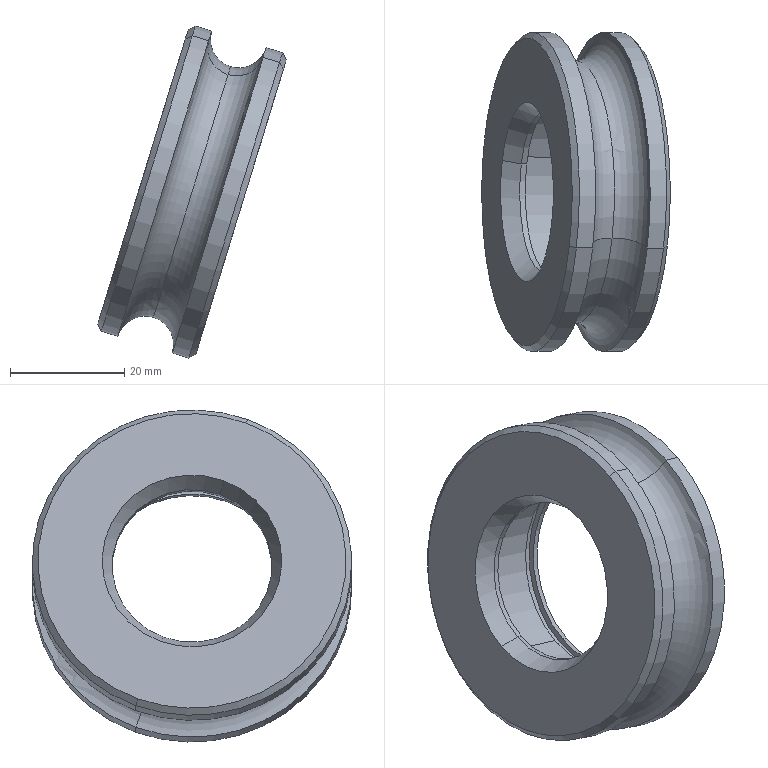Component | SolidWorks | DriveDevice-1_GuideWheelHub-1 | 1 solid | 27 faces | box 33.05 x 56 x 58.23 mm | volume 21349 mm3 | cylinder 12 | cone 6 | plane 5 | torus 4 | commonest cylinder face diameters 56 x4 35 x4 37 x2 28 x2
build123d program:
from build123d import *


with BuildPart() as part:
    # Sketch1 → Revolve1 (revolve)
    with BuildSketch(Plane(origin=(0, 0, 0), x_dir=(0, 0, -1), z_dir=(1, 0, 0)), mode=Mode.PRIVATE) as revolve1_sk:
        with BuildLine():
            Line((2.985, 14), (3.985, 14))
            Line((3.985, 14), (3.985, 17.5))
            Line((3.985, 17.5), (14.985, 17.5))
            Line((14.985, 17.5), (14.985, 18.5))
            Line((14.985, 18.5), (16.985, 18.5))
            Line((16.985, 18.5), (16.985, 17.5))
            Line((16.985, 17.5), (17.985, 17.5))
            Line((17.985, 17.5), (17.985, 27))
            Line((17.985, 27), (16.985, 28))
            Line((16.985, 28), (13.992, 28))
            ThreePointArc((13.992, 28), (8.992, 23), (3.992, 28))
            Line((3.992, 28), (1, 28))
            Line((1, 28), (0, 27))
            Line((0, 27), (0, 15.75))
            Line((0, 15.75), (2.985, 14))
        make_face()
    revolve(revolve1_sk.sketch.rotate(Axis((0, 0, 0), (0, 0, -1)), 90), axis=Axis((0, 0, 0), (0, 0, -1)))


solid = part.part

# Placed as in the assembly
solid = solid.moved(Location((-214.709, 15, 17.054), (0, -72.922, 83.044)))
STEP:
#1=COLOUR_RGB('',0.7922,0.8196,0.9333);
#2=FILL_AREA_STYLE_COLOUR('',#1);
#3=FILL_AREA_STYLE('',(#2));
#4=SURFACE_STYLE_FILL_AREA(#3);
#5=SURFACE_SIDE_STYLE('',(#4));
#6=SURFACE_STYLE_USAGE(.BOTH.,#5);
#7=PRESENTATION_STYLE_ASSIGNMENT((#6));
#8=CARTESIAN_POINT('',(-8.606,0.9787,-0.361));
#9=VERTEX_POINT('',#8);
#10=CARTESIAN_POINT('',(-8.364,0.9094,-0.2427));
#11=VERTEX_POINT('',#10);
#12=CARTESIAN_POINT('',(-8.418,0.9787,-0.4188));
#13=DIRECTION('',(0.1034,0.936,0.3366));
#14=DIRECTION('',(0.,-0.3384,0.941));
#15=AXIS2_PLACEMENT_3D('',#12,#13,#14);
#16=CIRCLE('',#15,0.1969);
#17=EDGE_CURVE('',#9,#11,#16,.T.);
#18=ORIENTED_EDGE('',*,*,#17,.T.);
#19=CARTESIAN_POINT('',(-7.866,0.2717,1.378));
#20=VERTEX_POINT('',#19);
#21=CARTESIAN_POINT('',(-8.115,0.5906,0.5675));
#22=DIRECTION('',(-0.9559,-0.,0.2937));
#23=DIRECTION('',(0.2937,0.,0.9559));
#24=AXIS2_PLACEMENT_3D('',#21,#22,#23);
#25=CIRCLE('',#24,0.9055);
#26=EDGE_CURVE('',#11,#20,#25,.T.);
#27=ORIENTED_EDGE('',*,*,#26,.T.);
#28=CARTESIAN_POINT('',(-8.,0.2024,1.612));
#29=VERTEX_POINT('',#28);
#30=CARTESIAN_POINT('',(-7.812,0.2024,1.554));
#31=DIRECTION('',(-0.1034,-0.936,-0.3366));
#32=DIRECTION('',(0.,0.3384,-0.941));
#33=AXIS2_PLACEMENT_3D('',#30,#31,#32);
#34=CIRCLE('',#33,0.1969);
#35=EDGE_CURVE('',#29,#20,#34,.T.);
#36=ORIENTED_EDGE('',*,*,#35,.F.);
#37=CARTESIAN_POINT('',(-8.303,0.5906,0.6253));
#38=DIRECTION('',(-0.9559,-0.,0.2937));
#39=DIRECTION('',(-0.2749,0.3521,-0.8947));
#40=AXIS2_PLACEMENT_3D('',#37,#38,#39);
#41=CIRCLE('',#40,1.102);
#42=EDGE_CURVE('',#9,#29,#41,.T.);
#43=ORIENTED_EDGE('',*,*,#42,.F.);
#44=EDGE_LOOP('',(#18,#27,#36,#43));
#45=FACE_OUTER_BOUND('',#44,.T.);
#46=CARTESIAN_POINT('',(-8.115,0.5906,0.5675));
#47=DIRECTION('',(-0.9559,-0.,0.2937));
#48=DIRECTION('',(-0.2749,0.3521,-0.8947));
#49=AXIS2_PLACEMENT_3D('',#46,#47,#48);
#50=TOROIDAL_SURFACE('',#49,1.102,0.1969);
#51=ADVANCED_FACE('',(#45),#50,.F.);
#52=ORIENTED_EDGE('',*,*,#35,.T.);
#53=CARTESIAN_POINT('',(-8.115,0.5906,0.5675));
#54=DIRECTION('',(-0.9559,-0.,0.2937));
#55=DIRECTION('',(0.2937,0.,0.9559));
#56=AXIS2_PLACEMENT_3D('',#53,#54,#55);
#57=CIRCLE('',#56,0.9055);
#58=EDGE_CURVE('',#20,#11,#57,.T.);
#59=ORIENTED_EDGE('',*,*,#58,.T.);
#60=ORIENTED_EDGE('',*,*,#17,.F.);
#61=CARTESIAN_POINT('',(-8.303,0.5906,0.6253));
#62=DIRECTION('',(-0.9559,-0.,0.2937));
#63=DIRECTION('',(-0.2749,0.3521,-0.8947));
#64=AXIS2_PLACEMENT_3D('',#61,#62,#63);
#65=CIRCLE('',#64,1.102);
#66=EDGE_CURVE('',#29,#9,#65,.T.);
#67=ORIENTED_EDGE('',*,*,#66,.F.);
#68=EDGE_LOOP('',(#52,#59,#60,#67));
#69=FACE_OUTER_BOUND('',#68,.T.);
#70=CARTESIAN_POINT('',(-8.115,0.5906,0.5675));
#71=DIRECTION('',(-0.9559,-0.,0.2937));
#72=DIRECTION('',(-0.2749,0.3521,-0.8947));
#73=AXIS2_PLACEMENT_3D('',#70,#71,#72);
#74=TOROIDAL_SURFACE('',#73,1.102,0.1969);
#75=ADVANCED_FACE('',(#69),#74,.F.);
#76=CARTESIAN_POINT('',(-8.745,0.9648,-0.2796));
#77=VERTEX_POINT('',#76);
#78=CARTESIAN_POINT('',(-8.161,0.2163,1.622));
#79=VERTEX_POINT('',#78);
#80=CARTESIAN_POINT('',(-8.453,0.5906,0.6714));
#81=DIRECTION('',(-0.9559,-0.,0.2937));
#82=DIRECTION('',(-0.2749,0.3521,-0.8947));
#83=AXIS2_PLACEMENT_3D('',#80,#81,#82);
#84=CIRCLE('',#83,1.063);
#85=EDGE_CURVE('',#77,#79,#84,.T.);
#86=ORIENTED_EDGE('',*,*,#85,.F.);
#87=CARTESIAN_POINT('',(-8.718,0.9787,-0.3264));
#88=VERTEX_POINT('',#87);
#89=CARTESIAN_POINT('',(-8.718,0.9787,-0.3264));
#90=DIRECTION('',(0.4816,0.249,-0.8403));
#91=VECTOR('',#90,39.37);
#92=LINE('',#89,#91);
#93=EDGE_CURVE('',#77,#88,#92,.T.);
#94=ORIENTED_EDGE('',*,*,#93,.T.);
#95=CARTESIAN_POINT('',(-8.112,0.2024,1.646));
#96=VERTEX_POINT('',#95);
#97=CARTESIAN_POINT('',(-8.415,0.5906,0.6599));
#98=DIRECTION('',(-0.9559,-0.,0.2937));
#99=DIRECTION('',(-0.2749,0.3521,-0.8947));
#100=AXIS2_PLACEMENT_3D('',#97,#98,#99);
#101=CIRCLE('',#100,1.102);
#102=EDGE_CURVE('',#88,#96,#101,.T.);
#103=ORIENTED_EDGE('',*,*,#102,.T.);
#104=CARTESIAN_POINT('',(-8.112,0.2024,1.646));
#105=DIRECTION('',(0.8703,-0.249,0.425));
#106=VECTOR('',#105,39.37);
#107=LINE('',#104,#106);
#108=EDGE_CURVE('',#79,#96,#107,.T.);
#109=ORIENTED_EDGE('',*,*,#108,.F.);
#110=EDGE_LOOP('',(#86,#94,#103,#109));
#111=FACE_OUTER_BOUND('',#110,.T.);
#112=CARTESIAN_POINT('',(-8.415,0.5906,0.6599));
#113=DIRECTION('',(0.9559,0.,-0.2937));
#114=DIRECTION('',(0.2749,-0.3521,0.8947));
#115=AXIS2_PLACEMENT_3D('',#112,#113,#114);
#116=CONICAL_SURFACE('',#115,1.102,0.7854);
#117=ADVANCED_FACE('',(#111),#116,.T.);
#118=ORIENTED_EDGE('',*,*,#42,.T.);
#119=CARTESIAN_POINT('',(-8.15,0.2024,1.658));
#120=DIRECTION('',(-0.9559,-0.,0.2937));
#121=VECTOR('',#120,39.37);
#122=LINE('',#119,#121);
#123=EDGE_CURVE('',#29,#96,#122,.T.);
#124=ORIENTED_EDGE('',*,*,#123,.T.);
#125=ORIENTED_EDGE('',*,*,#102,.F.);
#126=CARTESIAN_POINT('',(-8.756,0.9787,-0.3148));
#127=DIRECTION('',(-0.9559,-0.,0.2937));
#128=VECTOR('',#127,39.37);
#129=LINE('',#126,#128);
#130=EDGE_CURVE('',#9,#88,#129,.T.);
#131=ORIENTED_EDGE('',*,*,#130,.F.);
#132=EDGE_LOOP('',(#118,#124,#125,#131));
#133=FACE_OUTER_BOUND('',#132,.T.);
#134=CARTESIAN_POINT('',(-8.453,0.5906,0.6714));
#135=DIRECTION('',(-0.9559,-0.,0.2937));
#136=DIRECTION('',(-0.2749,0.3521,-0.8947));
#137=AXIS2_PLACEMENT_3D('',#134,#135,#136);
#138=CYLINDRICAL_SURFACE('',#137,1.102);
#139=ADVANCED_FACE('',(#133),#138,.T.);
#140=ORIENTED_EDGE('',*,*,#58,.F.);
#141=CARTESIAN_POINT('',(-7.624,0.2024,1.496));
#142=VERTEX_POINT('',#141);
#143=CARTESIAN_POINT('',(-7.812,0.2024,1.554));
#144=DIRECTION('',(-0.1034,-0.936,-0.3366));
#145=DIRECTION('',(0.,0.3384,-0.941));
#146=AXIS2_PLACEMENT_3D('',#143,#144,#145);
#147=CIRCLE('',#146,0.1969);
#148=EDGE_CURVE('',#20,#142,#147,.T.);
#149=ORIENTED_EDGE('',*,*,#148,.T.);
#150=CARTESIAN_POINT('',(-8.23,0.9787,-0.4766));
#151=VERTEX_POINT('',#150);
#152=CARTESIAN_POINT('',(-7.927,0.5906,0.5097));
#153=DIRECTION('',(-0.9559,-0.,0.2937));
#154=DIRECTION('',(-0.2749,0.3521,-0.8947));
#155=AXIS2_PLACEMENT_3D('',#152,#153,#154);
#156=CIRCLE('',#155,1.102);
#157=EDGE_CURVE('',#142,#151,#156,.T.);
#158=ORIENTED_EDGE('',*,*,#157,.T.);
#159=CARTESIAN_POINT('',(-8.418,0.9787,-0.4188));
#160=DIRECTION('',(0.1034,0.936,0.3366));
#161=DIRECTION('',(0.,-0.3384,0.941));
#162=AXIS2_PLACEMENT_3D('',#159,#160,#161);
#163=CIRCLE('',#162,0.1969);
#164=EDGE_CURVE('',#11,#151,#163,.T.);
#165=ORIENTED_EDGE('',*,*,#164,.F.);
#166=EDGE_LOOP('',(#140,#149,#158,#165));
#167=FACE_OUTER_BOUND('',#166,.T.);
#168=CARTESIAN_POINT('',(-8.115,0.5906,0.5675));
#169=DIRECTION('',(-0.9559,-0.,0.2937));
#170=DIRECTION('',(-0.2749,0.3521,-0.8947));
#171=AXIS2_PLACEMENT_3D('',#168,#169,#170);
#172=TOROIDAL_SURFACE('',#171,1.102,0.1969);
#173=ADVANCED_FACE('',(#167),#172,.F.);
#174=CARTESIAN_POINT('',(-8.117,0.9787,-0.5112));
#175=VERTEX_POINT('',#174);
#176=CARTESIAN_POINT('',(-7.511,0.2024,1.461));
#177=VERTEX_POINT('',#176);
#178=CARTESIAN_POINT('',(-7.814,0.5906,0.4751));
#179=DIRECTION('',(-0.9559,-0.,0.2937));
#180=DIRECTION('',(-0.2749,0.3521,-0.8947));
#181=AXIS2_PLACEMENT_3D('',#178,#179,#180);
#182=CIRCLE('',#181,1.102);
#183=EDGE_CURVE('',#175,#177,#182,.T.);
#184=ORIENTED_EDGE('',*,*,#183,.T.);
#185=CARTESIAN_POINT('',(-8.15,0.2024,1.658));
#186=DIRECTION('',(-0.9559,-0.,0.2937));
#187=VECTOR('',#186,39.37);
#188=LINE('',#185,#187);
#189=EDGE_CURVE('',#177,#142,#188,.T.);
#190=ORIENTED_EDGE('',*,*,#189,.T.);
#191=CARTESIAN_POINT('',(-7.927,0.5906,0.5097));
#192=DIRECTION('',(-0.9559,-0.,0.2937));
#193=DIRECTION('',(-0.2749,0.3521,-0.8947));
#194=AXIS2_PLACEMENT_3D('',#191,#192,#193);
#195=CIRCLE('',#194,1.102);
#196=EDGE_CURVE('',#151,#142,#195,.T.);
#197=ORIENTED_EDGE('',*,*,#196,.F.);
#198=CARTESIAN_POINT('',(-8.756,0.9787,-0.3148));
#199=DIRECTION('',(-0.9559,-0.,0.2937));
#200=VECTOR('',#199,39.37);
#201=LINE('',#198,#200);
#202=EDGE_CURVE('',#175,#151,#201,.T.);
#203=ORIENTED_EDGE('',*,*,#202,.F.);
#204=EDGE_LOOP('',(#184,#190,#197,#203));
#205=FACE_OUTER_BOUND('',#204,.T.);
#206=CARTESIAN_POINT('',(-8.453,0.5906,0.6714));
#207=DIRECTION('',(-0.9559,-0.,0.2937));
#208=DIRECTION('',(-0.2749,0.3521,-0.8947));
#209=AXIS2_PLACEMENT_3D('',#206,#207,#208);
#210=CYLINDRICAL_SURFACE('',#209,1.102);
#211=ADVANCED_FACE('',(#205),#210,.T.);
#212=CARTESIAN_POINT('',(-8.068,0.9648,-0.4876));
#213=VERTEX_POINT('',#212);
#214=CARTESIAN_POINT('',(-7.484,0.2163,1.415));
#215=VERTEX_POINT('',#214);
#216=CARTESIAN_POINT('',(-7.776,0.5906,0.4635));
#217=DIRECTION('',(-0.9559,-0.,0.2937));
#218=DIRECTION('',(-0.2749,0.3521,-0.8947));
#219=AXIS2_PLACEMENT_3D('',#216,#217,#218);
#220=CIRCLE('',#219,1.063);
#221=EDGE_CURVE('',#213,#215,#220,.T.);
#222=ORIENTED_EDGE('',*,*,#221,.T.);
#223=CARTESIAN_POINT('',(-7.484,0.2163,1.415));
#224=DIRECTION('',(-0.4816,-0.249,0.8403));
#225=VECTOR('',#224,39.37);
#226=LINE('',#223,#225);
#227=EDGE_CURVE('',#215,#177,#226,.T.);
#228=ORIENTED_EDGE('',*,*,#227,.T.);
#229=ORIENTED_EDGE('',*,*,#183,.F.);
#230=CARTESIAN_POINT('',(-8.068,0.9648,-0.4876));
#231=DIRECTION('',(-0.8703,0.249,-0.425));
#232=VECTOR('',#231,39.37);
#233=LINE('',#230,#232);
#234=EDGE_CURVE('',#213,#175,#233,.T.);
#235=ORIENTED_EDGE('',*,*,#234,.F.);
#236=EDGE_LOOP('',(#222,#228,#229,#235));
#237=FACE_OUTER_BOUND('',#236,.T.);
#238=CARTESIAN_POINT('',(-7.776,0.5906,0.4635));
#239=DIRECTION('',(-0.9559,-0.,0.2937));
#240=DIRECTION('',(-0.2749,0.3521,-0.8947));
#241=AXIS2_PLACEMENT_3D('',#238,#239,#240);
#242=CONICAL_SURFACE('',#241,1.063,0.7854);
#243=ADVANCED_FACE('',(#237),#242,.T.);
#244=CARTESIAN_POINT('',(-7.587,0.348,1.08));
#245=VERTEX_POINT('',#244);
#246=CARTESIAN_POINT('',(-7.966,0.8331,-0.1529));
#247=VERTEX_POINT('',#246);
#248=CARTESIAN_POINT('',(-7.776,0.5906,0.4635));
#249=DIRECTION('',(-0.9559,-0.,0.2937));
#250=DIRECTION('',(-0.2749,0.3521,-0.8947));
#251=AXIS2_PLACEMENT_3D('',#248,#249,#250);
#252=CIRCLE('',#251,0.689);
#253=EDGE_CURVE('',#245,#247,#252,.T.);
#254=ORIENTED_EDGE('',*,*,#253,.F.);
#255=CARTESIAN_POINT('',(-7.625,0.348,1.091));
#256=VERTEX_POINT('',#255);
#257=CARTESIAN_POINT('',(-8.264,0.348,1.288));
#258=DIRECTION('',(-0.9559,-0.,0.2937));
#259=VECTOR('',#258,39.37);
#260=LINE('',#257,#259);
#261=EDGE_CURVE('',#245,#256,#260,.T.);
#262=ORIENTED_EDGE('',*,*,#261,.T.);
#263=CARTESIAN_POINT('',(-8.003,0.8331,-0.1414));
#264=VERTEX_POINT('',#263);
#265=CARTESIAN_POINT('',(-7.814,0.5906,0.4751));
#266=DIRECTION('',(-0.9559,-0.,0.2937));
#267=DIRECTION('',(-0.2749,0.3521,-0.8947));
#268=AXIS2_PLACEMENT_3D('',#265,#266,#267);
#269=CIRCLE('',#268,0.689);
#270=EDGE_CURVE('',#256,#264,#269,.T.);
#271=ORIENTED_EDGE('',*,*,#270,.T.);
#272=CARTESIAN_POINT('',(-8.642,0.8331,0.05501));
#273=DIRECTION('',(-0.9559,-0.,0.2937));
#274=VECTOR('',#273,39.37);
#275=LINE('',#272,#274);
#276=EDGE_CURVE('',#247,#264,#275,.T.);
#277=ORIENTED_EDGE('',*,*,#276,.F.);
#278=EDGE_LOOP('',(#254,#262,#271,#277));
#279=FACE_OUTER_BOUND('',#278,.T.);
#280=CARTESIAN_POINT('',(-8.453,0.5906,0.6714));
#281=DIRECTION('',(-0.9559,-0.,0.2937));
#282=DIRECTION('',(-0.2749,0.3521,-0.8947));
#283=AXIS2_PLACEMENT_3D('',#280,#281,#282);
#284=CYLINDRICAL_SURFACE('',#283,0.689);
#285=ADVANCED_FACE('',(#279),#284,.F.);
#286=CARTESIAN_POINT('',(-7.614,0.3341,1.127));
#287=VERTEX_POINT('',#286);
#288=CARTESIAN_POINT('',(-8.014,0.847,-0.1766));
#289=VERTEX_POINT('',#288);
#290=CARTESIAN_POINT('',(-7.814,0.5906,0.4751));
#291=DIRECTION('',(-0.9559,-0.,0.2937));
#292=DIRECTION('',(-0.2749,0.3521,-0.8947));
#293=AXIS2_PLACEMENT_3D('',#290,#291,#292);
#294=CIRCLE('',#293,0.7283);
#295=EDGE_CURVE('',#287,#289,#294,.T.);
#296=ORIENTED_EDGE('',*,*,#295,.F.);
#297=CARTESIAN_POINT('',(-7.689,0.3341,1.15));
#298=VERTEX_POINT('',#297);
#299=CARTESIAN_POINT('',(-8.253,0.3341,1.323));
#300=DIRECTION('',(-0.9559,-0.,0.2937));
#301=VECTOR('',#300,39.37);
#302=LINE('',#299,#301);
#303=EDGE_CURVE('',#287,#298,#302,.T.);
#304=ORIENTED_EDGE('',*,*,#303,.T.);
#305=CARTESIAN_POINT('',(-8.089,0.847,-0.1535));
#306=VERTEX_POINT('',#305);
#307=CARTESIAN_POINT('',(-7.889,0.5906,0.4982));
#308=DIRECTION('',(-0.9559,-0.,0.2937));
#309=DIRECTION('',(-0.2749,0.3521,-0.8947));
#310=AXIS2_PLACEMENT_3D('',#307,#308,#309);
#311=CIRCLE('',#310,0.7283);
#312=EDGE_CURVE('',#298,#306,#311,.T.);
#313=ORIENTED_EDGE('',*,*,#312,.T.);
#314=CARTESIAN_POINT('',(-8.653,0.847,0.01979));
#315=DIRECTION('',(-0.9559,-0.,0.2937));
#316=VECTOR('',#315,39.37);
#317=LINE('',#314,#316);
#318=EDGE_CURVE('',#289,#306,#317,.T.);
#319=ORIENTED_EDGE('',*,*,#318,.F.);
#320=EDGE_LOOP('',(#296,#304,#313,#319));
#321=FACE_OUTER_BOUND('',#320,.T.);
#322=CARTESIAN_POINT('',(-8.453,0.5906,0.6714));
#323=DIRECTION('',(-0.9559,-0.,0.2937));
#324=DIRECTION('',(-0.2749,0.3521,-0.8947));
#325=AXIS2_PLACEMENT_3D('',#322,#323,#324);
#326=CYLINDRICAL_SURFACE('',#325,0.7283);
#327=ADVANCED_FACE('',(#321),#326,.F.);
#328=CARTESIAN_POINT('',(-7.7,0.348,1.115));
#329=VERTEX_POINT('',#328);
#330=CARTESIAN_POINT('',(-8.079,0.8331,-0.1182));
#331=VERTEX_POINT('',#330);
#332=CARTESIAN_POINT('',(-7.889,0.5906,0.4982));
#333=DIRECTION('',(-0.9559,-0.,0.2937));
#334=DIRECTION('',(-0.2749,0.3521,-0.8947));
#335=AXIS2_PLACEMENT_3D('',#332,#333,#334);
#336=CIRCLE('',#335,0.689);
#337=EDGE_CURVE('',#329,#331,#336,.T.);
#338=ORIENTED_EDGE('',*,*,#337,.F.);
#339=CARTESIAN_POINT('',(-8.114,0.348,1.242));
#340=VERTEX_POINT('',#339);
#341=CARTESIAN_POINT('',(-8.264,0.348,1.288));
#342=DIRECTION('',(-0.9559,-0.,0.2937));
#343=VECTOR('',#342,39.37);
#344=LINE('',#341,#343);
#345=EDGE_CURVE('',#329,#340,#344,.T.);
#346=ORIENTED_EDGE('',*,*,#345,.T.);
#347=CARTESIAN_POINT('',(-8.493,0.8331,0.008942));
#348=VERTEX_POINT('',#347);
#349=CARTESIAN_POINT('',(-8.303,0.5906,0.6254));
#350=DIRECTION('',(-0.9559,-0.,0.2937));
#351=DIRECTION('',(-0.2749,0.3521,-0.8947));
#352=AXIS2_PLACEMENT_3D('',#349,#350,#351);
#353=CIRCLE('',#352,0.689);
#354=EDGE_CURVE('',#340,#348,#353,.T.);
#355=ORIENTED_EDGE('',*,*,#354,.T.);
#356=CARTESIAN_POINT('',(-8.642,0.8331,0.05501));
#357=DIRECTION('',(-0.9559,-0.,0.2937));
#358=VECTOR('',#357,39.37);
#359=LINE('',#356,#358);
#360=EDGE_CURVE('',#331,#348,#359,.T.);
#361=ORIENTED_EDGE('',*,*,#360,.F.);
#362=EDGE_LOOP('',(#338,#346,#355,#361));
#363=FACE_OUTER_BOUND('',#362,.T.);
#364=CARTESIAN_POINT('',(-8.453,0.5906,0.6714));
#365=DIRECTION('',(-0.9559,-0.,0.2937));
#366=DIRECTION('',(-0.2749,0.3521,-0.8947));
#367=AXIS2_PLACEMENT_3D('',#364,#365,#366);
#368=CYLINDRICAL_SURFACE('',#367,0.689);
#369=ADVANCED_FACE('',(#363),#368,.F.);
#370=CARTESIAN_POINT('',(-8.152,0.3965,1.119));
#371=VERTEX_POINT('',#370);
#372=CARTESIAN_POINT('',(-8.455,0.7846,0.1322));
#373=VERTEX_POINT('',#372);
#374=CARTESIAN_POINT('',(-8.303,0.5906,0.6254));
#375=DIRECTION('',(-0.9559,-0.,0.2937));
#376=DIRECTION('',(-0.2749,0.3521,-0.8947));
#377=AXIS2_PLACEMENT_3D('',#374,#375,#376);
#378=CIRCLE('',#377,0.5512);
#379=EDGE_CURVE('',#371,#373,#378,.T.);
#380=ORIENTED_EDGE('',*,*,#379,.F.);
#381=CARTESIAN_POINT('',(-8.189,0.3965,1.13));
#382=VERTEX_POINT('',#381);
#383=CARTESIAN_POINT('',(-8.302,0.3965,1.165));
#384=DIRECTION('',(-0.9559,-0.,0.2937));
#385=VECTOR('',#384,39.37);
#386=LINE('',#383,#385);
#387=EDGE_CURVE('',#371,#382,#386,.T.);
#388=ORIENTED_EDGE('',*,*,#387,.T.);
#389=CARTESIAN_POINT('',(-8.492,0.7846,0.1438));
#390=VERTEX_POINT('',#389);
#391=CARTESIAN_POINT('',(-8.341,0.5906,0.6369));
#392=DIRECTION('',(-0.9559,-0.,0.2937));
#393=DIRECTION('',(-0.2749,0.3521,-0.8947));
#394=AXIS2_PLACEMENT_3D('',#391,#392,#393);
#395=CIRCLE('',#394,0.5512);
#396=EDGE_CURVE('',#382,#390,#395,.T.);
#397=ORIENTED_EDGE('',*,*,#396,.T.);
#398=CARTESIAN_POINT('',(-8.605,0.7846,0.1783));
#399=DIRECTION('',(-0.9559,-0.,0.2937));
#400=VECTOR('',#399,39.37);
#401=LINE('',#398,#400);
#402=EDGE_CURVE('',#373,#390,#401,.T.);
#403=ORIENTED_EDGE('',*,*,#402,.F.);
#404=EDGE_LOOP('',(#380,#388,#397,#403));
#405=FACE_OUTER_BOUND('',#404,.T.);
#406=CARTESIAN_POINT('',(-8.453,0.5906,0.6714));
#407=DIRECTION('',(-0.9559,-0.,0.2937));
#408=DIRECTION('',(-0.2749,0.3521,-0.8947));
#409=AXIS2_PLACEMENT_3D('',#406,#407,#408);
#410=CYLINDRICAL_SURFACE('',#409,0.5512);
#411=ADVANCED_FACE('',(#405),#410,.F.);
#412=ORIENTED_EDGE('',*,*,#396,.F.);
#413=CARTESIAN_POINT('',(-8.283,0.3722,1.226));
#414=VERTEX_POINT('',#413);
#415=CARTESIAN_POINT('',(-8.283,0.3722,1.226));
#416=DIRECTION('',(-0.6856,-0.1781,0.7059));
#417=VECTOR('',#416,39.37);
#418=LINE('',#415,#417);
#419=EDGE_CURVE('',#382,#414,#418,.T.);
#420=ORIENTED_EDGE('',*,*,#419,.T.);
#421=CARTESIAN_POINT('',(-8.624,0.8089,0.1167));
#422=VERTEX_POINT('',#421);
#423=CARTESIAN_POINT('',(-8.453,0.5906,0.6714));
#424=DIRECTION('',(-0.9559,-0.,0.2937));
#425=DIRECTION('',(-0.2749,0.3521,-0.8947));
#426=AXIS2_PLACEMENT_3D('',#423,#424,#425);
#427=CIRCLE('',#426,0.6201);
#428=EDGE_CURVE('',#414,#422,#427,.T.);
#429=ORIENTED_EDGE('',*,*,#428,.T.);
#430=CARTESIAN_POINT('',(-8.624,0.8089,0.1167));
#431=DIRECTION('',(-0.9636,0.1781,-0.1992));
#432=VECTOR('',#431,39.37);
#433=LINE('',#430,#432);
#434=EDGE_CURVE('',#390,#422,#433,.T.);
#435=ORIENTED_EDGE('',*,*,#434,.F.);
#436=EDGE_LOOP('',(#412,#420,#429,#435));
#437=FACE_OUTER_BOUND('',#436,.T.);
#438=CARTESIAN_POINT('',(-8.453,0.5906,0.6714));
#439=DIRECTION('',(-0.9559,-0.,0.2937));
#440=DIRECTION('',(-0.2749,0.3521,-0.8947));
#441=AXIS2_PLACEMENT_3D('',#438,#439,#440);
#442=CONICAL_SURFACE('',#441,0.6201,0.5303);
#443=ADVANCED_FACE('',(#437),#442,.F.);
#444=ORIENTED_EDGE('',*,*,#419,.F.);
#445=CARTESIAN_POINT('',(-8.341,0.5906,0.6369));
#446=DIRECTION('',(-0.9559,-0.,0.2937));
#447=DIRECTION('',(-0.2749,0.3521,-0.8947));
#448=AXIS2_PLACEMENT_3D('',#445,#446,#447);
#449=CIRCLE('',#448,0.5512);
#450=EDGE_CURVE('',#390,#382,#449,.T.);
#451=ORIENTED_EDGE('',*,*,#450,.F.);
#452=ORIENTED_EDGE('',*,*,#434,.T.);
#453=CARTESIAN_POINT('',(-8.453,0.5906,0.6714));
#454=DIRECTION('',(-0.9559,-0.,0.2937));
#455=DIRECTION('',(-0.2749,0.3521,-0.8947));
#456=AXIS2_PLACEMENT_3D('',#453,#454,#455);
#457=CIRCLE('',#456,0.6201);
#458=EDGE_CURVE('',#422,#414,#457,.T.);
#459=ORIENTED_EDGE('',*,*,#458,.T.);
#460=EDGE_LOOP('',(#444,#451,#452,#459));
#461=FACE_OUTER_BOUND('',#460,.T.);
#462=CARTESIAN_POINT('',(-8.453,0.5906,0.6714));
#463=DIRECTION('',(-0.9559,-0.,0.2937));
#464=DIRECTION('',(-0.2749,0.3521,-0.8947));
#465=AXIS2_PLACEMENT_3D('',#462,#463,#464);
#466=CONICAL_SURFACE('',#465,0.6201,0.5303);
#467=ADVANCED_FACE('',(#461),#466,.F.);
#468=ORIENTED_EDGE('',*,*,#387,.F.);
#469=CARTESIAN_POINT('',(-8.303,0.5906,0.6254));
#470=DIRECTION('',(-0.9559,-0.,0.2937));
#471=DIRECTION('',(-0.2749,0.3521,-0.8947));
#472=AXIS2_PLACEMENT_3D('',#469,#470,#471);
#473=CIRCLE('',#472,0.5512);
#474=EDGE_CURVE('',#373,#371,#473,.T.);
#475=ORIENTED_EDGE('',*,*,#474,.F.);
#476=ORIENTED_EDGE('',*,*,#402,.T.);
#477=ORIENTED_EDGE('',*,*,#450,.T.);
#478=EDGE_LOOP('',(#468,#475,#476,#477));
#479=FACE_OUTER_BOUND('',#478,.T.);
#480=CARTESIAN_POINT('',(-8.453,0.5906,0.6714));
#481=DIRECTION('',(-0.9559,-0.,0.2937));
#482=DIRECTION('',(-0.2749,0.3521,-0.8947));
#483=AXIS2_PLACEMENT_3D('',#480,#481,#482);
#484=CYLINDRICAL_SURFACE('',#483,0.5512);
#485=ADVANCED_FACE('',(#479),#484,.F.);
#486=CARTESIAN_POINT('',(-8.303,0.5906,0.6254));
#487=DIRECTION('',(-0.9559,-0.,0.2937));
#488=DIRECTION('',(-0.2749,0.3521,-0.8947));
#489=AXIS2_PLACEMENT_3D('',#486,#487,#488);
#490=CIRCLE('',#489,0.689);
#491=EDGE_CURVE('',#348,#340,#490,.T.);
#492=ORIENTED_EDGE('',*,*,#491,.F.);
#493=ORIENTED_EDGE('',*,*,#354,.F.);
#494=EDGE_LOOP('',(#492,#493));
#495=FACE_OUTER_BOUND('',#494,.T.);
#496=ORIENTED_EDGE('',*,*,#474,.T.);
#497=ORIENTED_EDGE('',*,*,#379,.T.);
#498=EDGE_LOOP('',(#496,#497));
#499=FACE_BOUND('',#498,.T.);
#500=CARTESIAN_POINT('',(-8.36,0.07467,0.4399));
#501=DIRECTION('',(-0.9559,-0.,0.2937));
#502=DIRECTION('',(-0.2749,0.3521,-0.8947));
#503=AXIS2_PLACEMENT_3D('',#500,#501,#502);
#504=PLANE('',#503);
#505=ADVANCED_FACE('',(#495,#499),#504,.F.);
#506=ORIENTED_EDGE('',*,*,#345,.F.);
#507=CARTESIAN_POINT('',(-7.889,0.5906,0.4982));
#508=DIRECTION('',(-0.9559,-0.,0.2937));
#509=DIRECTION('',(-0.2749,0.3521,-0.8947));
#510=AXIS2_PLACEMENT_3D('',#507,#508,#509);
#511=CIRCLE('',#510,0.689);
#512=EDGE_CURVE('',#331,#329,#511,.T.);
#513=ORIENTED_EDGE('',*,*,#512,.F.);
#514=ORIENTED_EDGE('',*,*,#360,.T.);
#515=ORIENTED_EDGE('',*,*,#491,.T.);
#516=EDGE_LOOP('',(#506,#513,#514,#515));
#517=FACE_OUTER_BOUND('',#516,.T.);
#518=CARTESIAN_POINT('',(-8.453,0.5906,0.6714));
#519=DIRECTION('',(-0.9559,-0.,0.2937));
#520=DIRECTION('',(-0.2749,0.3521,-0.8947));
#521=AXIS2_PLACEMENT_3D('',#518,#519,#520);
#522=CYLINDRICAL_SURFACE('',#521,0.689);
#523=ADVANCED_FACE('',(#517),#522,.F.);
#524=CARTESIAN_POINT('',(-7.889,0.5906,0.4982));
#525=DIRECTION('',(-0.9559,-0.,0.2937));
#526=DIRECTION('',(-0.2749,0.3521,-0.8947));
#527=AXIS2_PLACEMENT_3D('',#524,#525,#526);
#528=CIRCLE('',#527,0.7283);
#529=EDGE_CURVE('',#306,#298,#528,.T.);
#530=ORIENTED_EDGE('',*,*,#529,.F.);
#531=ORIENTED_EDGE('',*,*,#312,.F.);
#532=EDGE_LOOP('',(#530,#531));
#533=FACE_OUTER_BOUND('',#532,.T.);
#534=ORIENTED_EDGE('',*,*,#512,.T.);
#535=ORIENTED_EDGE('',*,*,#337,.T.);
#536=EDGE_LOOP('',(#534,#535));
#537=FACE_BOUND('',#536,.T.);
#538=CARTESIAN_POINT('',(-7.96,-0.05431,0.2663));
#539=DIRECTION('',(-0.9559,-0.,0.2937));
#540=DIRECTION('',(-0.2749,0.3521,-0.8947));
#541=AXIS2_PLACEMENT_3D('',#538,#539,#540);
#542=PLANE('',#541);
#543=ADVANCED_FACE('',(#533,#537),#542,.F.);
#544=ORIENTED_EDGE('',*,*,#303,.F.);
#545=CARTESIAN_POINT('',(-7.814,0.5906,0.4751));
#546=DIRECTION('',(-0.9559,-0.,0.2937));
#547=DIRECTION('',(-0.2749,0.3521,-0.8947));
#548=AXIS2_PLACEMENT_3D('',#545,#546,#547);
#549=CIRCLE('',#548,0.7283);
#550=EDGE_CURVE('',#289,#287,#549,.T.);
#551=ORIENTED_EDGE('',*,*,#550,.F.);
#552=ORIENTED_EDGE('',*,*,#318,.T.);
#553=ORIENTED_EDGE('',*,*,#529,.T.);
#554=EDGE_LOOP('',(#544,#551,#552,#553));
#555=FACE_OUTER_BOUND('',#554,.T.);
#556=CARTESIAN_POINT('',(-8.453,0.5906,0.6714));
#557=DIRECTION('',(-0.9559,-0.,0.2937));
#558=DIRECTION('',(-0.2749,0.3521,-0.8947));
#559=AXIS2_PLACEMENT_3D('',#556,#557,#558);
#560=CYLINDRICAL_SURFACE('',#559,0.7283);
#561=ADVANCED_FACE('',(#555),#560,.F.);
#562=CARTESIAN_POINT('',(-7.814,0.5906,0.4751));
#563=DIRECTION('',(-0.9559,-0.,0.2937));
#564=DIRECTION('',(-0.2749,0.3521,-0.8947));
#565=AXIS2_PLACEMENT_3D('',#562,#563,#564);
#566=CIRCLE('',#565,0.689);
#567=EDGE_CURVE('',#264,#256,#566,.T.);
#568=ORIENTED_EDGE('',*,*,#567,.F.);
#569=ORIENTED_EDGE('',*,*,#270,.F.);
#570=EDGE_LOOP('',(#568,#569));
#571=FACE_BOUND('',#570,.T.);
#572=ORIENTED_EDGE('',*,*,#550,.T.);
#573=ORIENTED_EDGE('',*,*,#295,.T.);
#574=EDGE_LOOP('',(#572,#573));
#575=FACE_OUTER_BOUND('',#574,.T.);
#576=CARTESIAN_POINT('',(-7.889,-0.09115,0.2299));
#577=DIRECTION('',(0.9559,0.,-0.2937));
#578=DIRECTION('',(0.2749,-0.3521,0.8947));
#579=AXIS2_PLACEMENT_3D('',#576,#577,#578);
#580=PLANE('',#579);
#581=ADVANCED_FACE('',(#571,#575),#580,.F.);
#582=ORIENTED_EDGE('',*,*,#261,.F.);
#583=CARTESIAN_POINT('',(-7.776,0.5906,0.4635));
#584=DIRECTION('',(-0.9559,-0.,0.2937));
#585=DIRECTION('',(-0.2749,0.3521,-0.8947));
#586=AXIS2_PLACEMENT_3D('',#583,#584,#585);
#587=CIRCLE('',#586,0.689);
#588=EDGE_CURVE('',#247,#245,#587,.T.);
#589=ORIENTED_EDGE('',*,*,#588,.F.);
#590=ORIENTED_EDGE('',*,*,#276,.T.);
#591=ORIENTED_EDGE('',*,*,#567,.T.);
#592=EDGE_LOOP('',(#582,#589,#590,#591));
#593=FACE_OUTER_BOUND('',#592,.T.);
#594=CARTESIAN_POINT('',(-8.453,0.5906,0.6714));
#595=DIRECTION('',(-0.9559,-0.,0.2937));
#596=DIRECTION('',(-0.2749,0.3521,-0.8947));
#597=AXIS2_PLACEMENT_3D('',#594,#595,#596);
#598=CYLINDRICAL_SURFACE('',#597,0.689);
#599=ADVANCED_FACE('',(#593),#598,.F.);
#600=ORIENTED_EDGE('',*,*,#221,.F.);
#601=CARTESIAN_POINT('',(-7.776,0.5906,0.4635));
#602=DIRECTION('',(-0.9559,-0.,0.2937));
#603=DIRECTION('',(-0.2749,0.3521,-0.8947));
#604=AXIS2_PLACEMENT_3D('',#601,#602,#603);
#605=CIRCLE('',#604,1.063);
#606=EDGE_CURVE('',#215,#213,#605,.T.);
#607=ORIENTED_EDGE('',*,*,#606,.F.);
#608=EDGE_LOOP('',(#600,#607));
#609=FACE_OUTER_BOUND('',#608,.T.);
#610=ORIENTED_EDGE('',*,*,#588,.T.);
#611=ORIENTED_EDGE('',*,*,#253,.T.);
#612=EDGE_LOOP('',(#610,#611));
#613=FACE_BOUND('',#612,.T.);
#614=CARTESIAN_POINT('',(-7.886,-0.4044,0.1057));
#615=DIRECTION('',(-0.9559,-0.,0.2937));
#616=DIRECTION('',(-0.2749,0.3521,-0.8947));
#617=AXIS2_PLACEMENT_3D('',#614,#615,#616);
#618=PLANE('',#617);
#619=ADVANCED_FACE('',(#609,#613),#618,.F.);
#620=ORIENTED_EDGE('',*,*,#227,.F.);
#621=ORIENTED_EDGE('',*,*,#606,.T.);
#622=ORIENTED_EDGE('',*,*,#234,.T.);
#623=CARTESIAN_POINT('',(-7.814,0.5906,0.4751));
#624=DIRECTION('',(-0.9559,-0.,0.2937));
#625=DIRECTION('',(-0.2749,0.3521,-0.8947));
#626=AXIS2_PLACEMENT_3D('',#623,#624,#625);
#627=CIRCLE('',#626,1.102);
#628=EDGE_CURVE('',#177,#175,#627,.T.);
#629=ORIENTED_EDGE('',*,*,#628,.F.);
#630=EDGE_LOOP('',(#620,#621,#622,#629));
#631=FACE_OUTER_BOUND('',#630,.T.);
#632=CARTESIAN_POINT('',(-7.776,0.5906,0.4635));
#633=DIRECTION('',(-0.9559,-0.,0.2937));
#634=DIRECTION('',(-0.2749,0.3521,-0.8947));
#635=AXIS2_PLACEMENT_3D('',#632,#633,#634);
#636=CONICAL_SURFACE('',#635,1.063,0.7854);
#637=ADVANCED_FACE('',(#631),#636,.T.);
#638=ORIENTED_EDGE('',*,*,#189,.F.);
#639=ORIENTED_EDGE('',*,*,#628,.T.);
#640=ORIENTED_EDGE('',*,*,#202,.T.);
#641=ORIENTED_EDGE('',*,*,#157,.F.);
#642=EDGE_LOOP('',(#638,#639,#640,#641));
#643=FACE_OUTER_BOUND('',#642,.T.);
#644=CARTESIAN_POINT('',(-8.453,0.5906,0.6714));
#645=DIRECTION('',(-0.9559,-0.,0.2937));
#646=DIRECTION('',(-0.2749,0.3521,-0.8947));
#647=AXIS2_PLACEMENT_3D('',#644,#645,#646);
#648=CYLINDRICAL_SURFACE('',#647,1.102);
#649=ADVANCED_FACE('',(#643),#648,.T.);
#650=ORIENTED_EDGE('',*,*,#26,.F.);
#651=ORIENTED_EDGE('',*,*,#164,.T.);
#652=ORIENTED_EDGE('',*,*,#196,.T.);
#653=ORIENTED_EDGE('',*,*,#148,.F.);
#654=EDGE_LOOP('',(#650,#651,#652,#653));
#655=FACE_OUTER_BOUND('',#654,.T.);
#656=CARTESIAN_POINT('',(-8.115,0.5906,0.5675));
#657=DIRECTION('',(-0.9559,-0.,0.2937));
#658=DIRECTION('',(-0.2749,0.3521,-0.8947));
#659=AXIS2_PLACEMENT_3D('',#656,#657,#658);
#660=TOROIDAL_SURFACE('',#659,1.102,0.1969);
#661=ADVANCED_FACE('',(#655),#660,.F.);
#662=ORIENTED_EDGE('',*,*,#123,.F.);
#663=ORIENTED_EDGE('',*,*,#66,.T.);
#664=ORIENTED_EDGE('',*,*,#130,.T.);
#665=CARTESIAN_POINT('',(-8.415,0.5906,0.6599));
#666=DIRECTION('',(-0.9559,-0.,0.2937));
#667=DIRECTION('',(-0.2749,0.3521,-0.8947));
#668=AXIS2_PLACEMENT_3D('',#665,#666,#667);
#669=CIRCLE('',#668,1.102);
#670=EDGE_CURVE('',#96,#88,#669,.T.);
#671=ORIENTED_EDGE('',*,*,#670,.F.);
#672=EDGE_LOOP('',(#662,#663,#664,#671));
#673=FACE_OUTER_BOUND('',#672,.T.);
#674=CARTESIAN_POINT('',(-8.453,0.5906,0.6714));
#675=DIRECTION('',(-0.9559,-0.,0.2937));
#676=DIRECTION('',(-0.2749,0.3521,-0.8947));
#677=AXIS2_PLACEMENT_3D('',#674,#675,#676);
#678=CYLINDRICAL_SURFACE('',#677,1.102);
#679=ADVANCED_FACE('',(#673),#678,.T.);
#680=ORIENTED_EDGE('',*,*,#93,.F.);
#681=CARTESIAN_POINT('',(-8.453,0.5906,0.6714));
#682=DIRECTION('',(-0.9559,-0.,0.2937));
#683=DIRECTION('',(-0.2749,0.3521,-0.8947));
#684=AXIS2_PLACEMENT_3D('',#681,#682,#683);
#685=CIRCLE('',#684,1.063);
#686=EDGE_CURVE('',#79,#77,#685,.T.);
#687=ORIENTED_EDGE('',*,*,#686,.F.);
#688=ORIENTED_EDGE('',*,*,#108,.T.);
#689=ORIENTED_EDGE('',*,*,#670,.T.);
#690=EDGE_LOOP('',(#680,#687,#688,#689));
#691=FACE_OUTER_BOUND('',#690,.T.);
#692=CARTESIAN_POINT('',(-8.415,0.5906,0.6599));
#693=DIRECTION('',(0.9559,0.,-0.2937));
#694=DIRECTION('',(0.2749,-0.3521,0.8947));
#695=AXIS2_PLACEMENT_3D('',#692,#693,#694);
#696=CONICAL_SURFACE('',#695,1.102,0.7854);
#697=ADVANCED_FACE('',(#691),#696,.T.);
#698=ORIENTED_EDGE('',*,*,#458,.F.);
#699=ORIENTED_EDGE('',*,*,#428,.F.);
#700=EDGE_LOOP('',(#698,#699));
#701=FACE_BOUND('',#700,.T.);
#702=ORIENTED_EDGE('',*,*,#686,.T.);
#703=ORIENTED_EDGE('',*,*,#85,.T.);
#704=EDGE_LOOP('',(#702,#703));
#705=FACE_OUTER_BOUND('',#704,.T.);
#706=CARTESIAN_POINT('',(-8.517,0.01018,0.4627));
#707=DIRECTION('',(0.9559,0.,-0.2937));
#708=DIRECTION('',(0.2749,-0.3521,0.8947));
#709=AXIS2_PLACEMENT_3D('',#706,#707,#708);
#710=PLANE('',#709);
#711=ADVANCED_FACE('',(#701,#705),#710,.F.);
#712=CLOSED_SHELL('',(#51,#75,#117,#139,#173,#211,#243,#285,#327,#369,#411,#443,#467,#485,#505,#523,#543,#561,#581,#599,#619,#637,#649,#661,#679,#697,#711));
#713=MANIFOLD_SOLID_BREP('',#712);
#714=STYLED_ITEM('',(#7),#713);
#715=PRESENTATION_LAYER_ASSIGNMENT('','',(#714));
#716=(LENGTH_UNIT()NAMED_UNIT(*)SI_UNIT($,.METRE.));
#717=LENGTH_MEASURE_WITH_UNIT(LENGTH_MEASURE(0.0254),#716);
#718=DIMENSIONAL_EXPONENTS(1.,0.,0.,0.,0.,0.,0.);
#719=(CONVERSION_BASED_UNIT('',#717)LENGTH_UNIT()NAMED_UNIT(#718));
#720=UNCERTAINTY_MEASURE_WITH_UNIT(LENGTH_MEASURE(0.00001),#719,'','');
#721=(NAMED_UNIT(*)PLANE_ANGLE_UNIT()SI_UNIT($,.RADIAN.));
#722=(NAMED_UNIT(*)SI_UNIT($,.STERADIAN.)SOLID_ANGLE_UNIT());
#723=(GEOMETRIC_REPRESENTATION_CONTEXT(3)GLOBAL_UNCERTAINTY_ASSIGNED_CONTEXT((#720))GLOBAL_UNIT_ASSIGNED_CONTEXT((#719,#721,#722))REPRESENTATION_CONTEXT('',''));
#724=MECHANICAL_DESIGN_GEOMETRIC_PRESENTATION_REPRESENTATION('',(#714),#723);
#725=CARTESIAN_POINT('',(0.,0.,0.));
#726=DIRECTION('',(0.,0.,1.));
#727=DIRECTION('',(1.,0.,0.));
#728=AXIS2_PLACEMENT_3D('',#725,#726,#727);
#729=(LENGTH_UNIT()NAMED_UNIT(*)SI_UNIT($,.METRE.));
#730=LENGTH_MEASURE_WITH_UNIT(LENGTH_MEASURE(0.0254),#729);
#731=DIMENSIONAL_EXPONENTS(1.,0.,0.,0.,0.,0.,0.);
#732=(CONVERSION_BASED_UNIT('',#730)LENGTH_UNIT()NAMED_UNIT(#731));
#733=UNCERTAINTY_MEASURE_WITH_UNIT(LENGTH_MEASURE(0.00001),#732,'','');
#734=(NAMED_UNIT(*)PLANE_ANGLE_UNIT()SI_UNIT($,.RADIAN.));
#735=(NAMED_UNIT(*)SI_UNIT($,.STERADIAN.)SOLID_ANGLE_UNIT());
#736=(GEOMETRIC_REPRESENTATION_CONTEXT(3)GLOBAL_UNCERTAINTY_ASSIGNED_CONTEXT((#733))GLOBAL_UNIT_ASSIGNED_CONTEXT((#732,#734,#735))REPRESENTATION_CONTEXT('',''));
#737=ADVANCED_BREP_SHAPE_REPRESENTATION('',(#713,#728),#736);